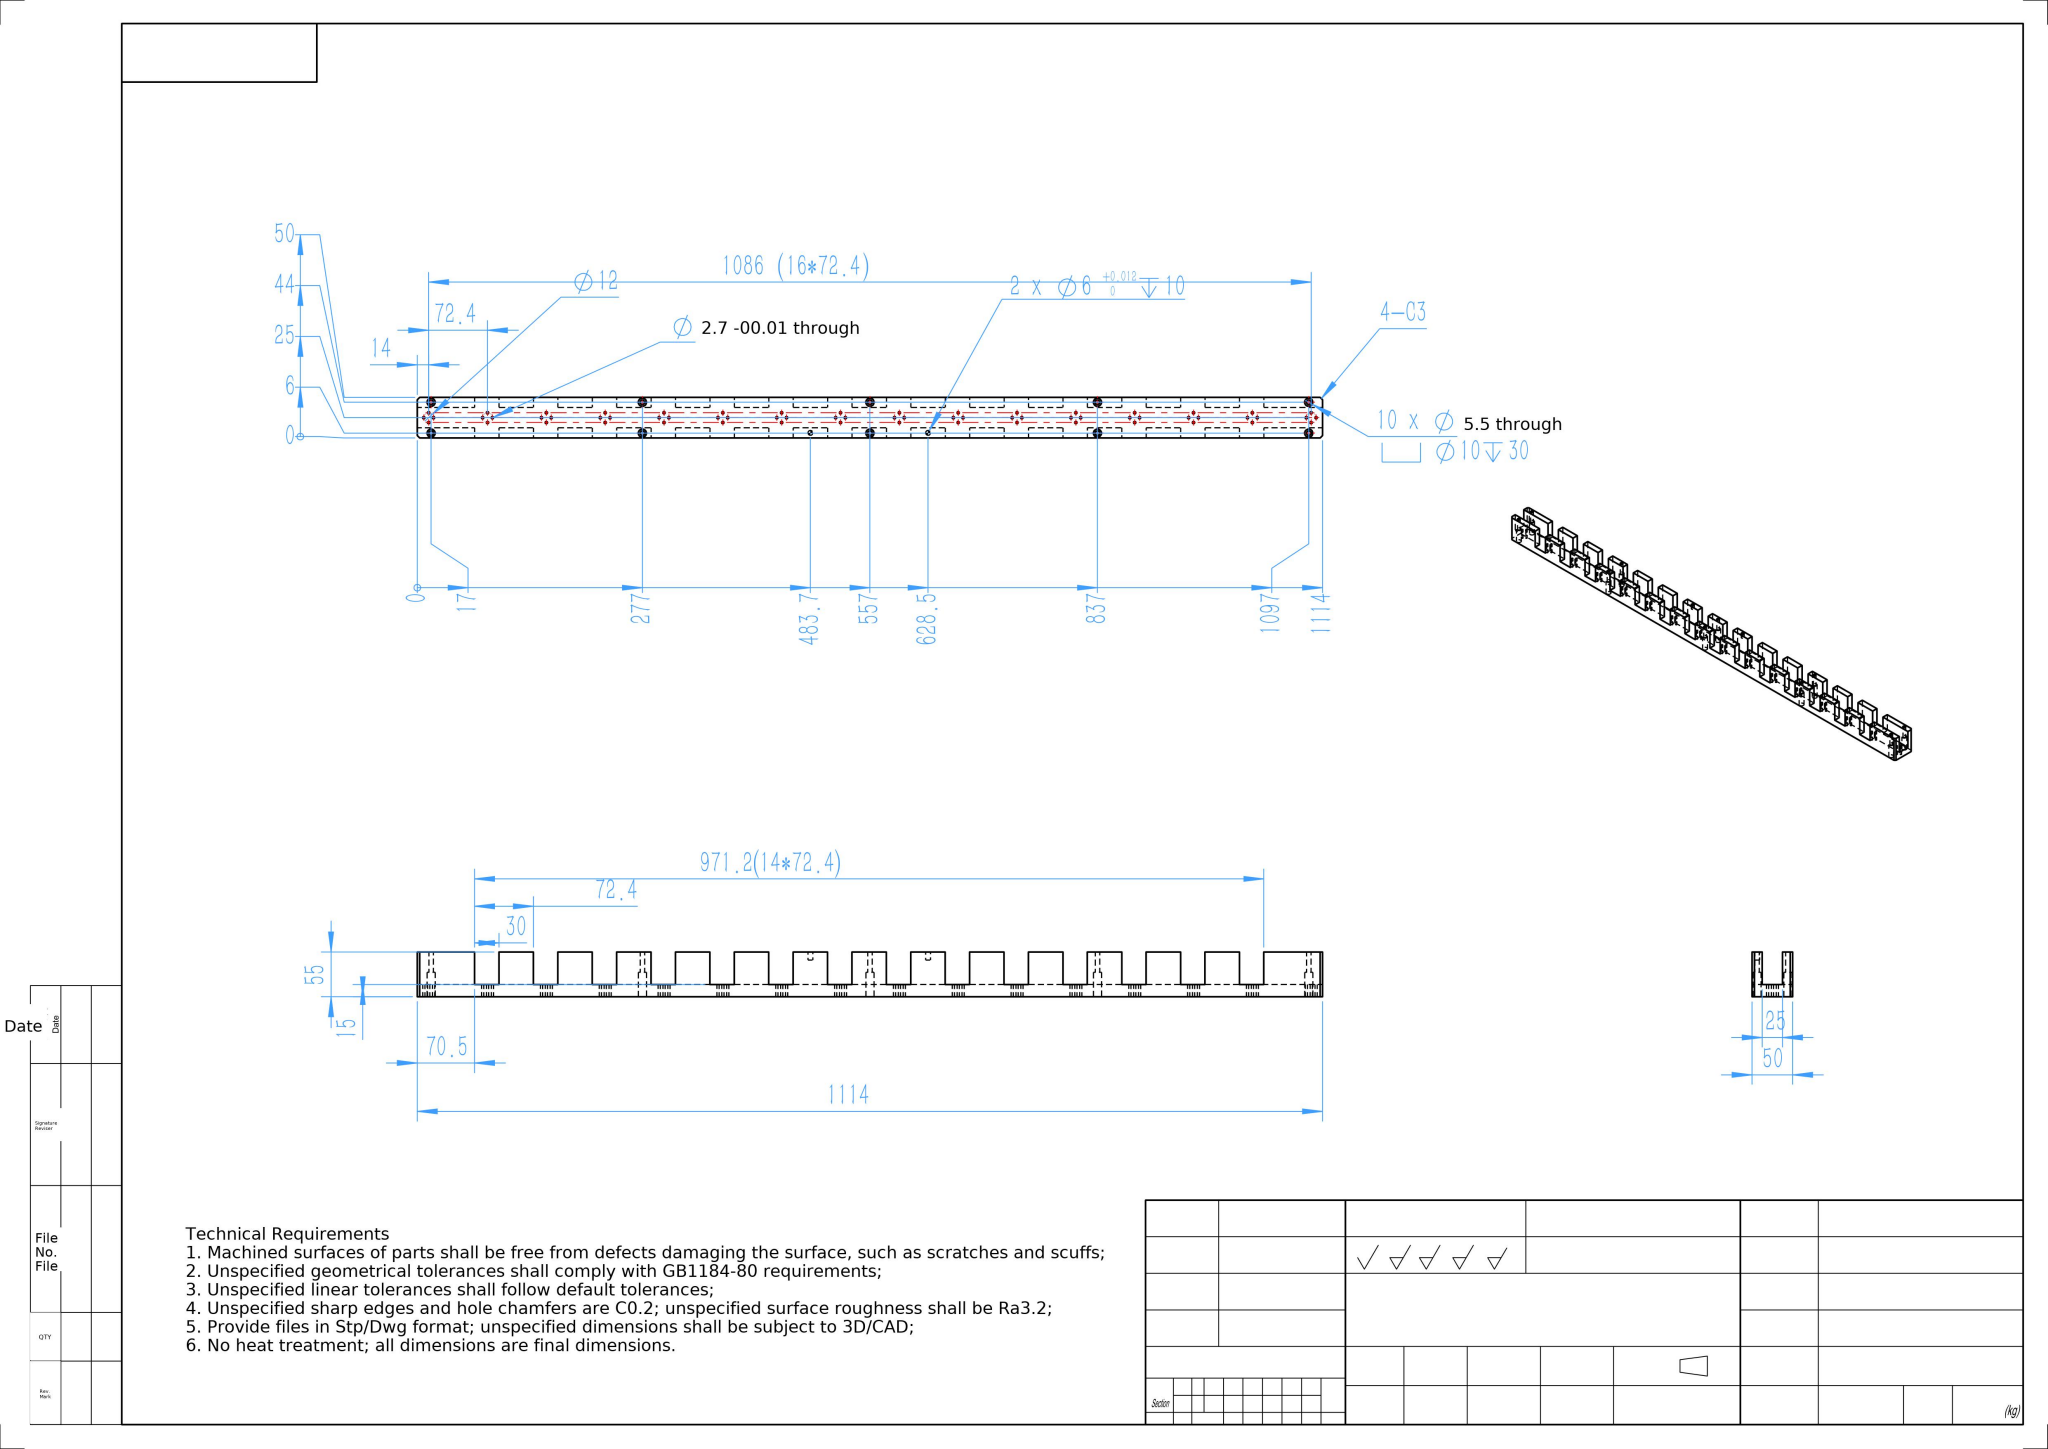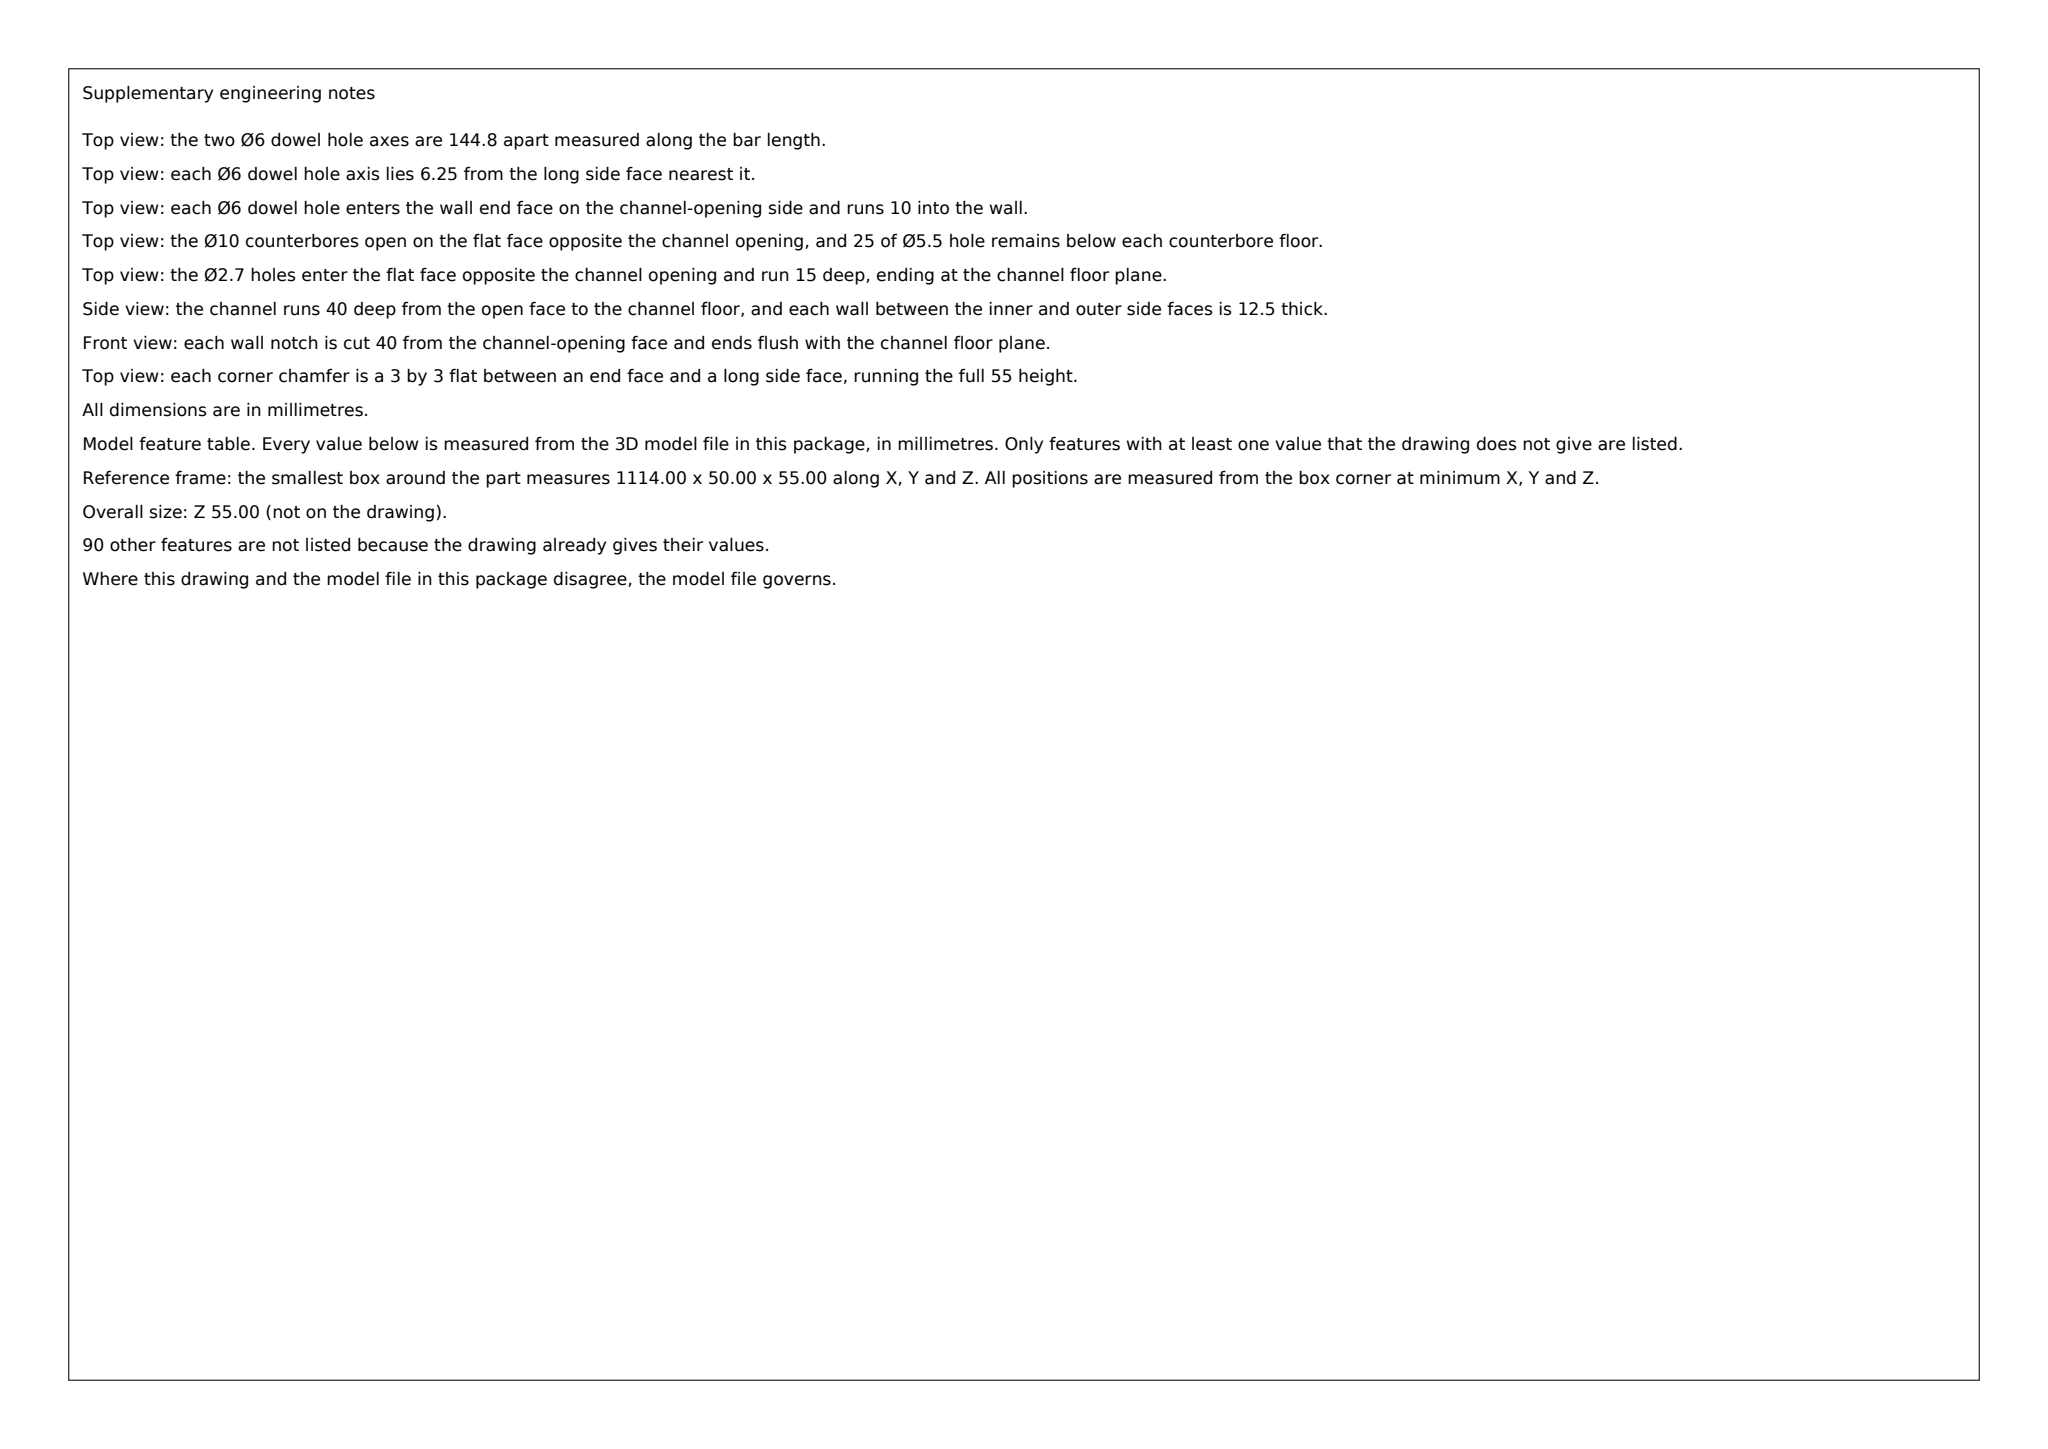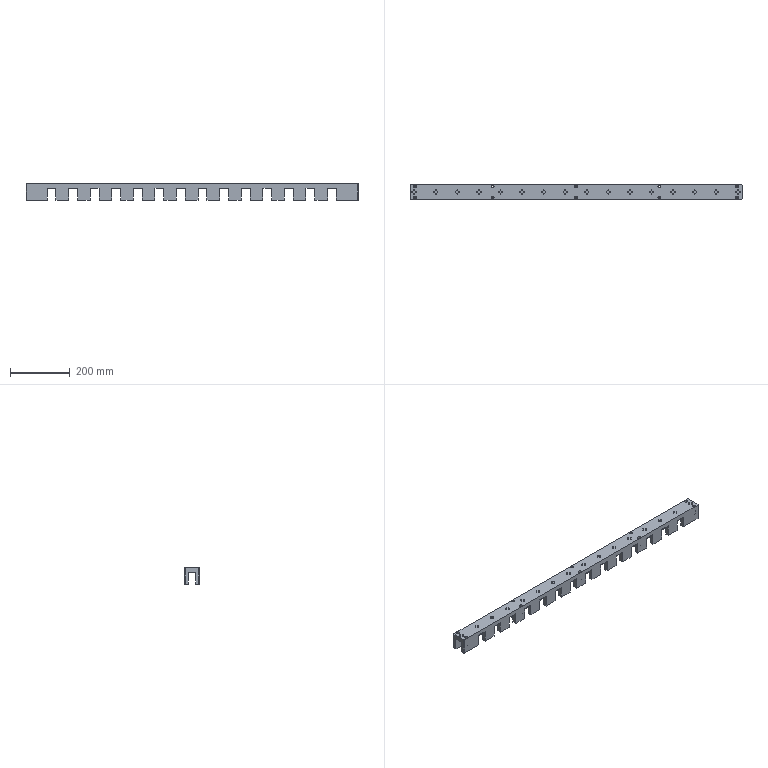Part | SolidWorks | mm | 1 solid | 310 faces | box 1114 x 50 x 55 mm | volume 1492946 mm3 | cylinder 172 | plane 138 | commonest cylinder face diameters 2.7 x128 10 x20 5.5 x20 6 x4
Drawing notes:
64X Ø2.7 THRU, 16 GRPS @72.4, GRP CL 14 FROM END; 4 HOLES ON Ø12 B.C., B.C. CL Y25 | from the solid: Ø2.7 z-holes x=8/14/14/20 repeating +72.4 to 1106 (64 total); y=19/25/31, i.e. ctr±6 and 25±6 => Ø12 B.C. centered 25 from bottom edge of 50 width
build123d program:
from build123d import *

# Parameters (mm, degrees)
SKETCH2_W                                       = 1114
SKETCH2_H                                       = 50
BOSS_EXTRUDE1_DEPTH                             = 70
M5_TAPPED_HOLE1_D                               = 4.2
M5_TAPPED_HOLE1_DEPTH                           = 12.4
M5_TAPPED_HOLE1_TIP                             = 1.262
CHAMFER1_SIZE                                   = 3
M5_TAPPED_HOLE2_D                               = 4.2
M5_TAPPED_HOLE2_DEPTH                           = 14
M5_TAPPED_HOLE2_TIP                             = 1.262
SKETCH10_W                                      = 15
SKETCH10_H                                      = 18
CUT_EXTRUDE1_DEPTH                              = 1117.477
SKETCH11_R                                      = 1.35
CUT_EXTRUDE2_DEPTH                              = 561.267
SKETCH13_W                                      = 40
SKETCH13_H                                      = 25
CUT_EXTRUDE4_DEPTH                              = 1117.477
SKETCH15_W                                      = 15
SKETCH15_H                                      = 16
CUT_EXTRUDE6_DEPTH                              = 1117.477
LPATTERN1_COUNT                                 = 16
LPATTERN1_PITCH                                 = 72.4
SKETCH16_W                                      = 30
SKETCH16_H                                      = 50
CUT_EXTRUDE7_DEPTH                              = 40
LPATTERN2_COUNT                                 = 14
LPATTERN2_PITCH                                 = 72.4
M5_HEX_SOCKET_HEAD_CAP_SCREW_CBORE1_D           = 5.5
M5_HEX_SOCKET_HEAD_CAP_SCREW_CBORE1_CBORE_D     = 10
M5_HEX_SOCKET_HEAD_CAP_SCREW_CBORE1_CBORE_DEPTH = 30
F_6_0MM_DOWEL_PIN_HOLE1_D                       = 6
F_6_0MM_DOWEL_PIN_HOLE1_DEPTH                   = 10


with BuildPart() as part:
    # Sketch2 → Boss-Extrude1 (new body)
    with BuildSketch(Plane.XY):
        Rectangle(SKETCH2_W, SKETCH2_H)
    extrude(amount=BOSS_EXTRUDE1_DEPTH)

    # M5 Tapped Hole1
    with Locations(Plane(origin=(0, 0, 0), x_dir=(1, 0, 0), z_dir=(0, 0, -1))):
        with Locations((550, 0), (-400, 0), (-550, 0), (400, 0)):
            Hole(M5_TAPPED_HOLE1_D / 2, depth=M5_TAPPED_HOLE1_DEPTH)
            with Locations((0, 0, -(M5_TAPPED_HOLE1_DEPTH + M5_TAPPED_HOLE1_TIP / 2))):  # 118° drill point
                Cone(0, M5_TAPPED_HOLE1_D / 2, M5_TAPPED_HOLE1_TIP, mode=Mode.SUBTRACT)

    # Chamfer1
    chamfer1_edges = [part.edges().sort_by_distance(p)[0] for p in [
        (557, -25, 35),
        (-557, -25, 35),
        (-557, 25, 35),
        (557, 25, 35),
    ]]
    chamfer(chamfer1_edges, length=CHAMFER1_SIZE)

    # M5 Tapped Hole2
    with Locations(Plane(origin=(0, 0, 0), x_dir=(-1, 0, 0), z_dir=(0, 0, -1))):
        with Locations((-350, 0), (0, 0), (350, 0)):
            Hole(M5_TAPPED_HOLE2_D / 2, depth=M5_TAPPED_HOLE2_DEPTH)
            with Locations((0, 0, -(M5_TAPPED_HOLE2_DEPTH + M5_TAPPED_HOLE2_TIP / 2))):  # 118° drill point
                Cone(0, M5_TAPPED_HOLE2_D / 2, M5_TAPPED_HOLE2_TIP, mode=Mode.SUBTRACT)

    # Sketch10 → Cut-Extrude1 (cut, through all)
    with BuildSketch(Plane.ZY.offset(557)):
        with Locations((62.5, 0)):
            Rectangle(SKETCH10_W, SKETCH10_H)
        with Locations((7.5, 0)):
            Rectangle(SKETCH10_W, SKETCH10_H)
    extrude(amount=-CUT_EXTRUDE1_DEPTH, mode=Mode.SUBTRACT)

    # Sketch11 → Cut-Extrude2 (cut, through all)
    with BuildSketch(Plane(origin=(0, 0, 15), x_dir=(-1, 0, 0), z_dir=(0, 0, -1))):
        with Locations((-543, 6)):
            Circle(SKETCH11_R)
        with Locations((-549, 0)):
            Circle(SKETCH11_R)
        with Locations((-537, 0)):
            Circle(SKETCH11_R)
        with Locations((-543, -6)):
            Circle(SKETCH11_R)
    cut_extrude2 = extrude(amount=-CUT_EXTRUDE2_DEPTH, mode=Mode.SUBTRACT)

    # Sketch13 → Cut-Extrude4 (cut, through all)
    with BuildSketch(Plane(origin=(557, 0, 0), x_dir=(0, 0, -1), z_dir=(1, 0, 0))):
        with Locations((-20, 0)):
            Rectangle(SKETCH13_W, SKETCH13_H)
    extrude(amount=-CUT_EXTRUDE4_DEPTH, mode=Mode.SUBTRACT)

    # Sketch15 → Cut-Extrude6 (cut, through all)
    with BuildSketch(Plane(origin=(557, 0, 0), x_dir=(0, 0, -1), z_dir=(1, 0, 0))):
        with Locations((-62.5, 17)):
            Rectangle(SKETCH15_W, SKETCH15_H)
        with Locations((-62.5, -17)):
            Rectangle(SKETCH15_W, SKETCH15_H)
    extrude(amount=-CUT_EXTRUDE6_DEPTH, mode=Mode.SUBTRACT)

    # LPattern1: Cut-Extrude2 ×16
    with Locations(*[(-i * LPATTERN1_PITCH, 0, 0) for i in range(1, LPATTERN1_COUNT)]):
        add(cut_extrude2, mode=Mode.SUBTRACT)

    # Sketch16 → Cut-Extrude7 (cut)
    with BuildSketch(Plane(origin=(0, 0, 0), x_dir=(-1, 0, 0), z_dir=(0, 0, -1))):
        with Locations((-469.7, 0)):
            Rectangle(SKETCH16_W, SKETCH16_H)
    cut_extrude7 = extrude(amount=-CUT_EXTRUDE7_DEPTH, mode=Mode.SUBTRACT)

    # LPattern2: Cut-Extrude7 ×14
    with Locations(*[(-i * LPATTERN2_PITCH, 0, 0) for i in range(1, LPATTERN2_COUNT)]):
        add(cut_extrude7, mode=Mode.SUBTRACT)

    # M5 Hex Socket Head Cap Screw CBORE1 (through all)
    with Locations(Plane.XY.offset(55)):
        with Locations((-540, -19), (-540, 19), (0, 19), (-280, 19), (280, 19), (540, 19), (540, -19), (280, -19), (-280, -19), (0, -19)):
            CounterBoreHole(M5_HEX_SOCKET_HEAD_CAP_SCREW_CBORE1_D / 2, M5_HEX_SOCKET_HEAD_CAP_SCREW_CBORE1_CBORE_D / 2, M5_HEX_SOCKET_HEAD_CAP_SCREW_CBORE1_CBORE_DEPTH)

    # 6.0mm Dowel Pin Hole1
    with Locations(Plane(origin=(0, 0, 0), x_dir=(-1, 0, 0), z_dir=(0, 0, -1))):
        with Locations((-71.5, -18.75), (73.3, -18.75)):
            Hole(F_6_0MM_DOWEL_PIN_HOLE1_D / 2, depth=F_6_0MM_DOWEL_PIN_HOLE1_DEPTH)


solid = part.part